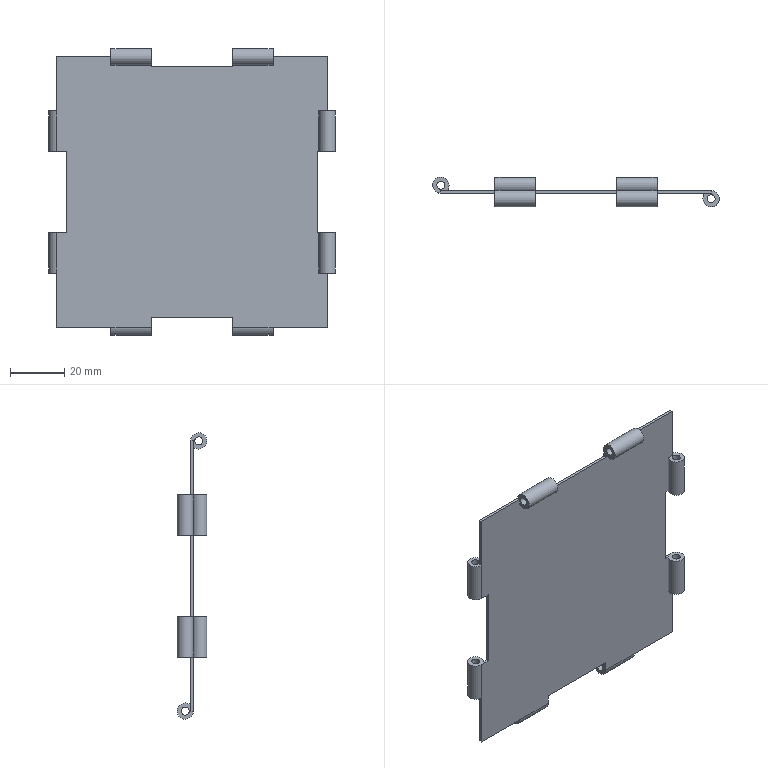Component | NX | PART_5 | 1 solid | 46 faces | volume 11939 mm3 | plane 30 | cylinder 16 | commonest cylinder face diameters 6 x8 3 x8